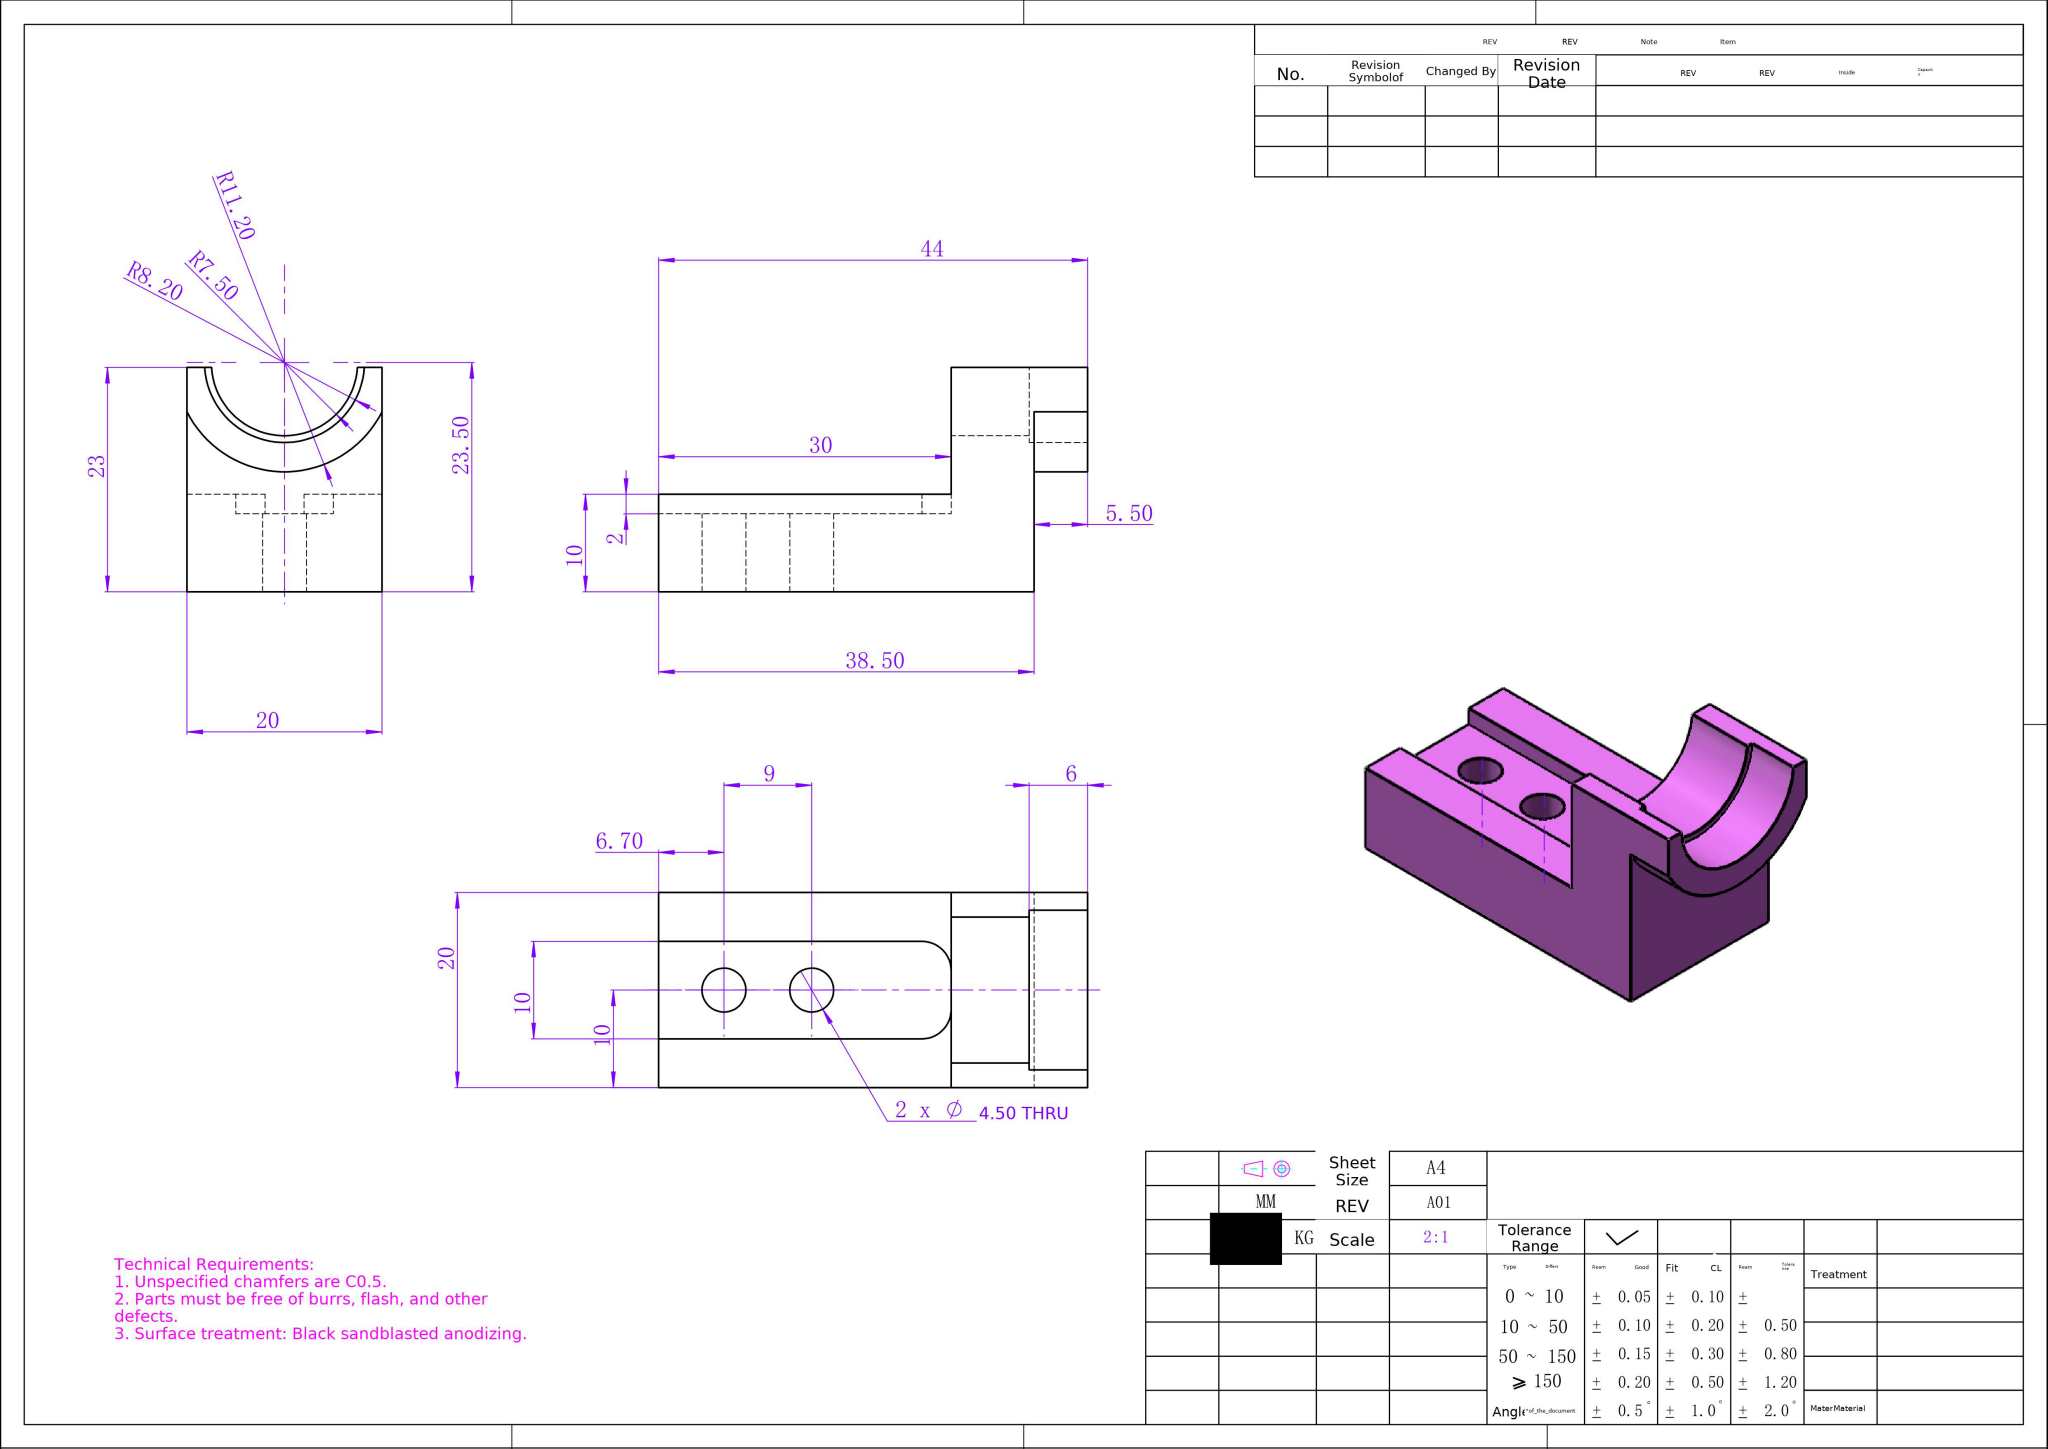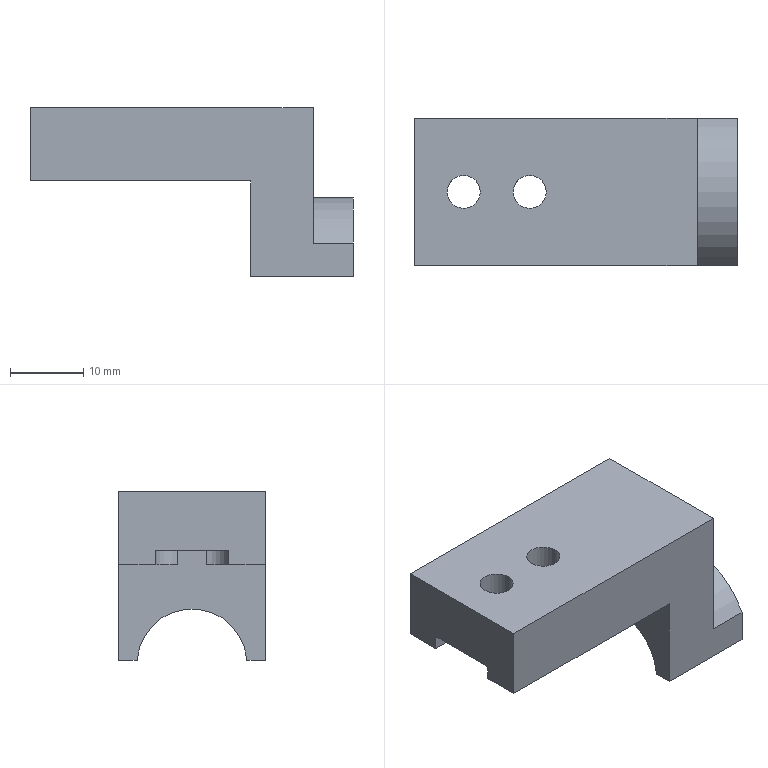Part | NX | mm | Dual-Bore Saddle Mounting Block | 1 solid | 24 faces | box 44 x 20 x 23 mm | volume 8816 mm3 | plane 15 | cylinder 9 | commonest cylinder face diameters 4.5 x4 6 x2 15 x1 16.4 x1 22.4 x1
STEP:
#1=COLOUR_RGB('',0.9529,0.498,1.);
#2=FILL_AREA_STYLE_COLOUR('',#1);
#3=FILL_AREA_STYLE('',(#2));
#4=SURFACE_STYLE_FILL_AREA(#3);
#5=SURFACE_SIDE_STYLE('',(#4));
#6=SURFACE_STYLE_USAGE(.BOTH.,#5);
#7=PRESENTATION_STYLE_ASSIGNMENT((#6));
#8=CARTESIAN_POINT('',(78.871,2.029,15.5));
#9=VERTEX_POINT('',#8);
#10=CARTESIAN_POINT('',(83.371,2.029,15.5));
#11=VERTEX_POINT('',#10);
#12=CARTESIAN_POINT('',(81.121,2.029,15.5));
#13=DIRECTION('',(0.,0.,1.));
#14=DIRECTION('',(-1.,0.,0.));
#15=AXIS2_PLACEMENT_3D('',#12,#13,#14);
#16=CIRCLE('',#15,2.25);
#17=EDGE_CURVE('',#9,#11,#16,.T.);
#18=ORIENTED_EDGE('',*,*,#17,.F.);
#19=CARTESIAN_POINT('',(78.871,2.029,23.5));
#20=VERTEX_POINT('',#19);
#21=CARTESIAN_POINT('',(78.871,2.029,23.5));
#22=DIRECTION('',(0.,0.,1.));
#23=VECTOR('',#22,1000.);
#24=LINE('',#21,#23);
#25=EDGE_CURVE('',#9,#20,#24,.T.);
#26=ORIENTED_EDGE('',*,*,#25,.T.);
#27=CARTESIAN_POINT('',(83.371,2.029,23.5));
#28=VERTEX_POINT('',#27);
#29=CARTESIAN_POINT('',(81.121,2.029,23.5));
#30=DIRECTION('',(0.,0.,1.));
#31=DIRECTION('',(1.,0.,0.));
#32=AXIS2_PLACEMENT_3D('',#29,#30,#31);
#33=CIRCLE('',#32,2.25);
#34=EDGE_CURVE('',#20,#28,#33,.T.);
#35=ORIENTED_EDGE('',*,*,#34,.T.);
#36=CARTESIAN_POINT('',(83.371,2.029,23.5));
#37=DIRECTION('',(0.,0.,1.));
#38=VECTOR('',#37,1000.);
#39=LINE('',#36,#38);
#40=EDGE_CURVE('',#11,#28,#39,.T.);
#41=ORIENTED_EDGE('',*,*,#40,.F.);
#42=EDGE_LOOP('',(#18,#26,#35,#41));
#43=FACE_OUTER_BOUND('',#42,.T.);
#44=CARTESIAN_POINT('',(81.121,2.029,23.5));
#45=DIRECTION('',(0.,0.,1.));
#46=DIRECTION('',(1.,0.,0.));
#47=AXIS2_PLACEMENT_3D('',#44,#45,#46);
#48=CYLINDRICAL_SURFACE('',#47,2.25);
#49=ADVANCED_FACE('',(#43),#48,.F.);
#50=CARTESIAN_POINT('',(87.871,2.029,15.5));
#51=VERTEX_POINT('',#50);
#52=CARTESIAN_POINT('',(92.371,2.029,15.5));
#53=VERTEX_POINT('',#52);
#54=CARTESIAN_POINT('',(90.121,2.029,15.5));
#55=DIRECTION('',(0.,0.,1.));
#56=DIRECTION('',(-1.,0.,0.));
#57=AXIS2_PLACEMENT_3D('',#54,#55,#56);
#58=CIRCLE('',#57,2.25);
#59=EDGE_CURVE('',#51,#53,#58,.T.);
#60=ORIENTED_EDGE('',*,*,#59,.F.);
#61=CARTESIAN_POINT('',(87.871,2.029,23.5));
#62=VERTEX_POINT('',#61);
#63=CARTESIAN_POINT('',(87.871,2.029,23.5));
#64=DIRECTION('',(0.,0.,1.));
#65=VECTOR('',#64,1000.);
#66=LINE('',#63,#65);
#67=EDGE_CURVE('',#51,#62,#66,.T.);
#68=ORIENTED_EDGE('',*,*,#67,.T.);
#69=CARTESIAN_POINT('',(92.371,2.029,23.5));
#70=VERTEX_POINT('',#69);
#71=CARTESIAN_POINT('',(90.121,2.029,23.5));
#72=DIRECTION('',(0.,0.,1.));
#73=DIRECTION('',(1.,0.,0.));
#74=AXIS2_PLACEMENT_3D('',#71,#72,#73);
#75=CIRCLE('',#74,2.25);
#76=EDGE_CURVE('',#62,#70,#75,.T.);
#77=ORIENTED_EDGE('',*,*,#76,.T.);
#78=CARTESIAN_POINT('',(92.371,2.029,23.5));
#79=DIRECTION('',(0.,0.,1.));
#80=VECTOR('',#79,1000.);
#81=LINE('',#78,#80);
#82=EDGE_CURVE('',#53,#70,#81,.T.);
#83=ORIENTED_EDGE('',*,*,#82,.F.);
#84=EDGE_LOOP('',(#60,#68,#77,#83));
#85=FACE_OUTER_BOUND('',#84,.T.);
#86=CARTESIAN_POINT('',(90.121,2.029,23.5));
#87=DIRECTION('',(0.,0.,1.));
#88=DIRECTION('',(1.,0.,0.));
#89=AXIS2_PLACEMENT_3D('',#86,#87,#88);
#90=CYLINDRICAL_SURFACE('',#89,2.25);
#91=ADVANCED_FACE('',(#85),#90,.F.);
#92=CARTESIAN_POINT('',(90.121,2.029,23.5));
#93=DIRECTION('',(0.,0.,1.));
#94=DIRECTION('',(1.,0.,0.));
#95=AXIS2_PLACEMENT_3D('',#92,#93,#94);
#96=CIRCLE('',#95,2.25);
#97=EDGE_CURVE('',#70,#62,#96,.T.);
#98=ORIENTED_EDGE('',*,*,#97,.F.);
#99=ORIENTED_EDGE('',*,*,#76,.F.);
#100=EDGE_LOOP('',(#98,#99));
#101=FACE_BOUND('',#100,.T.);
#102=CARTESIAN_POINT('',(81.121,2.029,23.5));
#103=DIRECTION('',(0.,0.,1.));
#104=DIRECTION('',(1.,0.,0.));
#105=AXIS2_PLACEMENT_3D('',#102,#103,#104);
#106=CIRCLE('',#105,2.25);
#107=EDGE_CURVE('',#28,#20,#106,.T.);
#108=ORIENTED_EDGE('',*,*,#107,.F.);
#109=ORIENTED_EDGE('',*,*,#34,.F.);
#110=EDGE_LOOP('',(#108,#109));
#111=FACE_BOUND('',#110,.T.);
#112=CARTESIAN_POINT('',(112.921,12.029,23.5));
#113=VERTEX_POINT('',#112);
#114=CARTESIAN_POINT('',(112.921,-7.971,23.5));
#115=VERTEX_POINT('',#114);
#116=CARTESIAN_POINT('',(112.921,12.029,23.5));
#117=DIRECTION('',(0.,-1.,0.));
#118=VECTOR('',#117,1000.);
#119=LINE('',#116,#118);
#120=EDGE_CURVE('',#113,#115,#119,.T.);
#121=ORIENTED_EDGE('',*,*,#120,.F.);
#122=CARTESIAN_POINT('',(74.421,12.029,23.5));
#123=VERTEX_POINT('',#122);
#124=CARTESIAN_POINT('',(74.421,12.029,23.5));
#125=DIRECTION('',(-1.,-0.,0.));
#126=VECTOR('',#125,1000.);
#127=LINE('',#124,#126);
#128=EDGE_CURVE('',#113,#123,#127,.T.);
#129=ORIENTED_EDGE('',*,*,#128,.T.);
#130=CARTESIAN_POINT('',(74.421,-7.971,23.5));
#131=VERTEX_POINT('',#130);
#132=CARTESIAN_POINT('',(74.421,-7.971,23.5));
#133=DIRECTION('',(0.,-1.,0.));
#134=VECTOR('',#133,1000.);
#135=LINE('',#132,#134);
#136=EDGE_CURVE('',#123,#131,#135,.T.);
#137=ORIENTED_EDGE('',*,*,#136,.T.);
#138=CARTESIAN_POINT('',(74.421,-7.971,23.5));
#139=DIRECTION('',(1.,0.,0.));
#140=VECTOR('',#139,1000.);
#141=LINE('',#138,#140);
#142=EDGE_CURVE('',#131,#115,#141,.T.);
#143=ORIENTED_EDGE('',*,*,#142,.T.);
#144=EDGE_LOOP('',(#121,#129,#137,#143));
#145=FACE_OUTER_BOUND('',#144,.T.);
#146=CARTESIAN_POINT('',(0.,0.,23.5));
#147=DIRECTION('',(0.,0.,-1.));
#148=DIRECTION('',(-1.,0.,0.));
#149=AXIS2_PLACEMENT_3D('',#146,#147,#148);
#150=PLANE('',#149);
#151=ADVANCED_FACE('',(#101,#111,#145),#150,.F.);
#152=CARTESIAN_POINT('',(104.421,-5.454,0.5));
#153=VERTEX_POINT('',#152);
#154=CARTESIAN_POINT('',(104.421,9.513,0.5));
#155=VERTEX_POINT('',#154);
#156=CARTESIAN_POINT('',(104.421,2.029,0.));
#157=DIRECTION('',(-1.,-0.,0.));
#158=DIRECTION('',(0.,-1.,0.));
#159=AXIS2_PLACEMENT_3D('',#156,#157,#158);
#160=CIRCLE('',#159,7.5);
#161=EDGE_CURVE('',#153,#155,#160,.T.);
#162=ORIENTED_EDGE('',*,*,#161,.T.);
#163=CARTESIAN_POINT('',(112.421,9.513,0.5));
#164=VERTEX_POINT('',#163);
#165=CARTESIAN_POINT('',(118.421,9.513,0.5));
#166=DIRECTION('',(1.,0.,0.));
#167=VECTOR('',#166,1000.);
#168=LINE('',#165,#167);
#169=EDGE_CURVE('',#155,#164,#168,.T.);
#170=ORIENTED_EDGE('',*,*,#169,.T.);
#171=CARTESIAN_POINT('',(112.421,-5.454,0.5));
#172=VERTEX_POINT('',#171);
#173=CARTESIAN_POINT('',(112.421,2.029,0.));
#174=DIRECTION('',(-1.,0.,0.));
#175=DIRECTION('',(0.,0.,-1.));
#176=AXIS2_PLACEMENT_3D('',#173,#174,#175);
#177=CIRCLE('',#176,7.5);
#178=EDGE_CURVE('',#172,#164,#177,.T.);
#179=ORIENTED_EDGE('',*,*,#178,.F.);
#180=CARTESIAN_POINT('',(118.421,-5.454,0.5));
#181=DIRECTION('',(-1.,-0.,0.));
#182=VECTOR('',#181,1000.);
#183=LINE('',#180,#182);
#184=EDGE_CURVE('',#172,#153,#183,.T.);
#185=ORIENTED_EDGE('',*,*,#184,.T.);
#186=EDGE_LOOP('',(#162,#170,#179,#185));
#187=FACE_OUTER_BOUND('',#186,.T.);
#188=CARTESIAN_POINT('',(118.421,2.029,0.));
#189=DIRECTION('',(-1.,-0.,0.));
#190=DIRECTION('',(0.,-1.,0.));
#191=AXIS2_PLACEMENT_3D('',#188,#189,#190);
#192=CYLINDRICAL_SURFACE('',#191,7.5);
#193=ADVANCED_FACE('',(#187),#192,.F.);
#194=CARTESIAN_POINT('',(74.421,-7.971,13.5));
#195=VERTEX_POINT('',#194);
#196=CARTESIAN_POINT('',(74.421,-2.971,13.5));
#197=VERTEX_POINT('',#196);
#198=CARTESIAN_POINT('',(74.421,-7.971,13.5));
#199=DIRECTION('',(-0.,1.,0.));
#200=VECTOR('',#199,1000.);
#201=LINE('',#198,#200);
#202=EDGE_CURVE('',#195,#197,#201,.T.);
#203=ORIENTED_EDGE('',*,*,#202,.T.);
#204=CARTESIAN_POINT('',(101.421,-2.971,13.5));
#205=VERTEX_POINT('',#204);
#206=CARTESIAN_POINT('',(74.421,-2.971,13.5));
#207=DIRECTION('',(-1.,0.,0.));
#208=VECTOR('',#207,1000.);
#209=LINE('',#206,#208);
#210=EDGE_CURVE('',#205,#197,#209,.T.);
#211=ORIENTED_EDGE('',*,*,#210,.F.);
#212=CARTESIAN_POINT('',(104.421,0.02923,13.5));
#213=VERTEX_POINT('',#212);
#214=CARTESIAN_POINT('',(101.421,0.02923,13.5));
#215=DIRECTION('',(0.,0.,-1.));
#216=DIRECTION('',(-1.,0.,0.));
#217=AXIS2_PLACEMENT_3D('',#214,#215,#216);
#218=CIRCLE('',#217,3.);
#219=EDGE_CURVE('',#213,#205,#218,.T.);
#220=ORIENTED_EDGE('',*,*,#219,.F.);
#221=CARTESIAN_POINT('',(104.421,-7.971,13.5));
#222=VERTEX_POINT('',#221);
#223=CARTESIAN_POINT('',(104.421,-7.971,13.5));
#224=DIRECTION('',(-0.,1.,0.));
#225=VECTOR('',#224,1000.);
#226=LINE('',#223,#225);
#227=EDGE_CURVE('',#222,#213,#226,.T.);
#228=ORIENTED_EDGE('',*,*,#227,.F.);
#229=CARTESIAN_POINT('',(74.421,-7.971,13.5));
#230=DIRECTION('',(1.,0.,0.));
#231=VECTOR('',#230,1000.);
#232=LINE('',#229,#231);
#233=EDGE_CURVE('',#195,#222,#232,.T.);
#234=ORIENTED_EDGE('',*,*,#233,.F.);
#235=EDGE_LOOP('',(#203,#211,#220,#228,#234));
#236=FACE_OUTER_BOUND('',#235,.T.);
#237=CARTESIAN_POINT('',(74.421,-7.971,13.5));
#238=DIRECTION('',(0.,0.,1.));
#239=DIRECTION('',(1.,0.,0.));
#240=AXIS2_PLACEMENT_3D('',#237,#238,#239);
#241=PLANE('',#240);
#242=ADVANCED_FACE('',(#236),#241,.F.);
#243=ORIENTED_EDGE('',*,*,#67,.F.);
#244=CARTESIAN_POINT('',(90.121,2.029,15.5));
#245=DIRECTION('',(0.,0.,1.));
#246=DIRECTION('',(-1.,0.,0.));
#247=AXIS2_PLACEMENT_3D('',#244,#245,#246);
#248=CIRCLE('',#247,2.25);
#249=EDGE_CURVE('',#53,#51,#248,.T.);
#250=ORIENTED_EDGE('',*,*,#249,.F.);
#251=ORIENTED_EDGE('',*,*,#82,.T.);
#252=ORIENTED_EDGE('',*,*,#97,.T.);
#253=EDGE_LOOP('',(#243,#250,#251,#252));
#254=FACE_OUTER_BOUND('',#253,.T.);
#255=CARTESIAN_POINT('',(90.121,2.029,23.5));
#256=DIRECTION('',(0.,0.,1.));
#257=DIRECTION('',(1.,0.,0.));
#258=AXIS2_PLACEMENT_3D('',#255,#256,#257);
#259=CYLINDRICAL_SURFACE('',#258,2.25);
#260=ADVANCED_FACE('',(#254),#259,.F.);
#261=ORIENTED_EDGE('',*,*,#25,.F.);
#262=CARTESIAN_POINT('',(81.121,2.029,15.5));
#263=DIRECTION('',(0.,0.,1.));
#264=DIRECTION('',(-1.,0.,0.));
#265=AXIS2_PLACEMENT_3D('',#262,#263,#264);
#266=CIRCLE('',#265,2.25);
#267=EDGE_CURVE('',#11,#9,#266,.T.);
#268=ORIENTED_EDGE('',*,*,#267,.F.);
#269=ORIENTED_EDGE('',*,*,#40,.T.);
#270=ORIENTED_EDGE('',*,*,#107,.T.);
#271=EDGE_LOOP('',(#261,#268,#269,#270));
#272=FACE_OUTER_BOUND('',#271,.T.);
#273=CARTESIAN_POINT('',(81.121,2.029,23.5));
#274=DIRECTION('',(0.,0.,1.));
#275=DIRECTION('',(1.,0.,0.));
#276=AXIS2_PLACEMENT_3D('',#273,#274,#275);
#277=CYLINDRICAL_SURFACE('',#276,2.25);
#278=ADVANCED_FACE('',(#272),#277,.F.);
#279=CARTESIAN_POINT('',(118.421,-7.971,5.044));
#280=VERTEX_POINT('',#279);
#281=CARTESIAN_POINT('',(118.421,-7.971,0.5));
#282=VERTEX_POINT('',#281);
#283=CARTESIAN_POINT('',(118.421,-7.971,23.5));
#284=DIRECTION('',(0.,0.,-1.));
#285=VECTOR('',#284,1000.);
#286=LINE('',#283,#285);
#287=EDGE_CURVE('',#280,#282,#286,.T.);
#288=ORIENTED_EDGE('',*,*,#287,.T.);
#289=CARTESIAN_POINT('',(118.421,-6.156,0.5));
#290=VERTEX_POINT('',#289);
#291=CARTESIAN_POINT('',(118.421,-7.971,0.5));
#292=DIRECTION('',(0.,1.,0.));
#293=VECTOR('',#292,1000.);
#294=LINE('',#291,#293);
#295=EDGE_CURVE('',#282,#290,#294,.T.);
#296=ORIENTED_EDGE('',*,*,#295,.T.);
#297=CARTESIAN_POINT('',(118.421,10.214,0.5));
#298=VERTEX_POINT('',#297);
#299=CARTESIAN_POINT('',(118.421,2.029,0.));
#300=DIRECTION('',(1.,0.,0.));
#301=DIRECTION('',(0.,0.,-1.));
#302=AXIS2_PLACEMENT_3D('',#299,#300,#301);
#303=CIRCLE('',#302,8.2);
#304=EDGE_CURVE('',#298,#290,#303,.T.);
#305=ORIENTED_EDGE('',*,*,#304,.F.);
#306=CARTESIAN_POINT('',(118.421,12.029,0.5));
#307=VERTEX_POINT('',#306);
#308=CARTESIAN_POINT('',(118.421,-7.971,0.5));
#309=DIRECTION('',(0.,1.,0.));
#310=VECTOR('',#309,1000.);
#311=LINE('',#308,#310);
#312=EDGE_CURVE('',#298,#307,#311,.T.);
#313=ORIENTED_EDGE('',*,*,#312,.T.);
#314=CARTESIAN_POINT('',(118.421,12.029,5.044));
#315=VERTEX_POINT('',#314);
#316=CARTESIAN_POINT('',(118.421,12.029,23.5));
#317=DIRECTION('',(0.,0.,-1.));
#318=VECTOR('',#317,1000.);
#319=LINE('',#316,#318);
#320=EDGE_CURVE('',#315,#307,#319,.T.);
#321=ORIENTED_EDGE('',*,*,#320,.F.);
#322=CARTESIAN_POINT('',(118.421,2.029,0.));
#323=DIRECTION('',(-1.,0.,0.));
#324=DIRECTION('',(0.,0.,-1.));
#325=AXIS2_PLACEMENT_3D('',#322,#323,#324);
#326=CIRCLE('',#325,11.2);
#327=EDGE_CURVE('',#280,#315,#326,.T.);
#328=ORIENTED_EDGE('',*,*,#327,.F.);
#329=EDGE_LOOP('',(#288,#296,#305,#313,#321,#328));
#330=FACE_OUTER_BOUND('',#329,.T.);
#331=CARTESIAN_POINT('',(118.421,-7.971,23.5));
#332=DIRECTION('',(-1.,0.,0.));
#333=DIRECTION('',(0.,0.,1.));
#334=AXIS2_PLACEMENT_3D('',#331,#332,#333);
#335=PLANE('',#334);
#336=ADVANCED_FACE('',(#330),#335,.F.);
#337=ORIENTED_EDGE('',*,*,#320,.T.);
#338=CARTESIAN_POINT('',(104.421,12.029,0.5));
#339=VERTEX_POINT('',#338);
#340=CARTESIAN_POINT('',(118.421,12.029,0.5));
#341=DIRECTION('',(-1.,-0.,0.));
#342=VECTOR('',#341,1000.);
#343=LINE('',#340,#342);
#344=EDGE_CURVE('',#307,#339,#343,.T.);
#345=ORIENTED_EDGE('',*,*,#344,.T.);
#346=CARTESIAN_POINT('',(104.421,12.029,13.5));
#347=VERTEX_POINT('',#346);
#348=CARTESIAN_POINT('',(104.421,12.029,0.));
#349=DIRECTION('',(0.,0.,-1.));
#350=VECTOR('',#349,1000.);
#351=LINE('',#348,#350);
#352=EDGE_CURVE('',#347,#339,#351,.T.);
#353=ORIENTED_EDGE('',*,*,#352,.F.);
#354=CARTESIAN_POINT('',(74.421,12.029,13.5));
#355=VERTEX_POINT('',#354);
#356=CARTESIAN_POINT('',(74.421,12.029,13.5));
#357=DIRECTION('',(1.,0.,0.));
#358=VECTOR('',#357,1000.);
#359=LINE('',#356,#358);
#360=EDGE_CURVE('',#355,#347,#359,.T.);
#361=ORIENTED_EDGE('',*,*,#360,.F.);
#362=CARTESIAN_POINT('',(74.421,12.029,23.5));
#363=DIRECTION('',(0.,0.,-1.));
#364=VECTOR('',#363,1000.);
#365=LINE('',#362,#364);
#366=EDGE_CURVE('',#123,#355,#365,.T.);
#367=ORIENTED_EDGE('',*,*,#366,.F.);
#368=ORIENTED_EDGE('',*,*,#128,.F.);
#369=CARTESIAN_POINT('',(112.921,12.029,5.044));
#370=VERTEX_POINT('',#369);
#371=CARTESIAN_POINT('',(112.921,12.029,23.5));
#372=DIRECTION('',(0.,0.,1.));
#373=VECTOR('',#372,1000.);
#374=LINE('',#371,#373);
#375=EDGE_CURVE('',#370,#113,#374,.T.);
#376=ORIENTED_EDGE('',*,*,#375,.F.);
#377=CARTESIAN_POINT('',(112.921,12.029,5.044));
#378=DIRECTION('',(1.,0.,0.));
#379=VECTOR('',#378,1000.);
#380=LINE('',#377,#379);
#381=EDGE_CURVE('',#370,#315,#380,.T.);
#382=ORIENTED_EDGE('',*,*,#381,.T.);
#383=EDGE_LOOP('',(#337,#345,#353,#361,#367,#368,#376,#382));
#384=FACE_OUTER_BOUND('',#383,.T.);
#385=CARTESIAN_POINT('',(74.421,12.029,23.5));
#386=DIRECTION('',(0.,-1.,0.));
#387=DIRECTION('',(1.,0.,0.));
#388=AXIS2_PLACEMENT_3D('',#385,#386,#387);
#389=PLANE('',#388);
#390=ADVANCED_FACE('',(#384),#389,.F.);
#391=CARTESIAN_POINT('',(74.421,-2.971,15.5));
#392=VERTEX_POINT('',#391);
#393=CARTESIAN_POINT('',(74.421,7.029,15.5));
#394=VERTEX_POINT('',#393);
#395=CARTESIAN_POINT('',(74.421,7.029,15.5));
#396=DIRECTION('',(0.,1.,0.));
#397=VECTOR('',#396,1000.);
#398=LINE('',#395,#397);
#399=EDGE_CURVE('',#392,#394,#398,.T.);
#400=ORIENTED_EDGE('',*,*,#399,.F.);
#401=CARTESIAN_POINT('',(74.421,-2.971,15.5));
#402=DIRECTION('',(0.,0.,-1.));
#403=VECTOR('',#402,1000.);
#404=LINE('',#401,#403);
#405=EDGE_CURVE('',#392,#197,#404,.T.);
#406=ORIENTED_EDGE('',*,*,#405,.T.);
#407=ORIENTED_EDGE('',*,*,#202,.F.);
#408=CARTESIAN_POINT('',(74.421,-7.971,23.5));
#409=DIRECTION('',(0.,0.,-1.));
#410=VECTOR('',#409,1000.);
#411=LINE('',#408,#410);
#412=EDGE_CURVE('',#131,#195,#411,.T.);
#413=ORIENTED_EDGE('',*,*,#412,.F.);
#414=ORIENTED_EDGE('',*,*,#136,.F.);
#415=ORIENTED_EDGE('',*,*,#366,.T.);
#416=CARTESIAN_POINT('',(74.421,7.029,13.5));
#417=VERTEX_POINT('',#416);
#418=CARTESIAN_POINT('',(74.421,-7.971,13.5));
#419=DIRECTION('',(-0.,1.,0.));
#420=VECTOR('',#419,1000.);
#421=LINE('',#418,#420);
#422=EDGE_CURVE('',#417,#355,#421,.T.);
#423=ORIENTED_EDGE('',*,*,#422,.F.);
#424=CARTESIAN_POINT('',(74.421,7.029,15.5));
#425=DIRECTION('',(0.,0.,-1.));
#426=VECTOR('',#425,1000.);
#427=LINE('',#424,#426);
#428=EDGE_CURVE('',#394,#417,#427,.T.);
#429=ORIENTED_EDGE('',*,*,#428,.F.);
#430=EDGE_LOOP('',(#400,#406,#407,#413,#414,#415,#423,#429));
#431=FACE_OUTER_BOUND('',#430,.T.);
#432=CARTESIAN_POINT('',(74.421,-7.971,23.5));
#433=DIRECTION('',(1.,0.,0.));
#434=DIRECTION('',(0.,0.,-1.));
#435=AXIS2_PLACEMENT_3D('',#432,#433,#434);
#436=PLANE('',#435);
#437=ADVANCED_FACE('',(#431),#436,.F.);
#438=CARTESIAN_POINT('',(104.421,-7.971,0.5));
#439=VERTEX_POINT('',#438);
#440=CARTESIAN_POINT('',(104.421,-7.971,0.));
#441=DIRECTION('',(0.,0.,-1.));
#442=VECTOR('',#441,1000.);
#443=LINE('',#440,#442);
#444=EDGE_CURVE('',#222,#439,#443,.T.);
#445=ORIENTED_EDGE('',*,*,#444,.T.);
#446=CARTESIAN_POINT('',(118.421,-7.971,0.5));
#447=DIRECTION('',(-1.,-0.,0.));
#448=VECTOR('',#447,1000.);
#449=LINE('',#446,#448);
#450=EDGE_CURVE('',#282,#439,#449,.T.);
#451=ORIENTED_EDGE('',*,*,#450,.F.);
#452=ORIENTED_EDGE('',*,*,#287,.F.);
#453=CARTESIAN_POINT('',(112.921,-7.971,5.044));
#454=VERTEX_POINT('',#453);
#455=CARTESIAN_POINT('',(112.921,-7.971,5.044));
#456=DIRECTION('',(1.,0.,0.));
#457=VECTOR('',#456,1000.);
#458=LINE('',#455,#457);
#459=EDGE_CURVE('',#454,#280,#458,.T.);
#460=ORIENTED_EDGE('',*,*,#459,.F.);
#461=CARTESIAN_POINT('',(112.921,-7.971,23.5));
#462=DIRECTION('',(0.,0.,-1.));
#463=VECTOR('',#462,1000.);
#464=LINE('',#461,#463);
#465=EDGE_CURVE('',#115,#454,#464,.T.);
#466=ORIENTED_EDGE('',*,*,#465,.F.);
#467=ORIENTED_EDGE('',*,*,#142,.F.);
#468=ORIENTED_EDGE('',*,*,#412,.T.);
#469=ORIENTED_EDGE('',*,*,#233,.T.);
#470=EDGE_LOOP('',(#445,#451,#452,#460,#466,#467,#468,#469));
#471=FACE_OUTER_BOUND('',#470,.T.);
#472=CARTESIAN_POINT('',(74.421,-7.971,23.5));
#473=DIRECTION('',(0.,1.,0.));
#474=DIRECTION('',(0.,0.,1.));
#475=AXIS2_PLACEMENT_3D('',#472,#473,#474);
#476=PLANE('',#475);
#477=ADVANCED_FACE('',(#471),#476,.F.);
#478=ORIENTED_EDGE('',*,*,#352,.T.);
#479=CARTESIAN_POINT('',(104.421,-7.971,0.5));
#480=DIRECTION('',(0.,1.,0.));
#481=VECTOR('',#480,1000.);
#482=LINE('',#479,#481);
#483=EDGE_CURVE('',#155,#339,#482,.T.);
#484=ORIENTED_EDGE('',*,*,#483,.F.);
#485=ORIENTED_EDGE('',*,*,#161,.F.);
#486=CARTESIAN_POINT('',(104.421,-7.971,0.5));
#487=DIRECTION('',(0.,1.,0.));
#488=VECTOR('',#487,1000.);
#489=LINE('',#486,#488);
#490=EDGE_CURVE('',#439,#153,#489,.T.);
#491=ORIENTED_EDGE('',*,*,#490,.F.);
#492=ORIENTED_EDGE('',*,*,#444,.F.);
#493=ORIENTED_EDGE('',*,*,#227,.T.);
#494=CARTESIAN_POINT('',(104.421,0.02923,15.5));
#495=VERTEX_POINT('',#494);
#496=CARTESIAN_POINT('',(104.421,0.02923,15.5));
#497=DIRECTION('',(0.,0.,-1.));
#498=VECTOR('',#497,1000.);
#499=LINE('',#496,#498);
#500=EDGE_CURVE('',#495,#213,#499,.T.);
#501=ORIENTED_EDGE('',*,*,#500,.F.);
#502=CARTESIAN_POINT('',(104.421,4.029,15.5));
#503=VERTEX_POINT('',#502);
#504=CARTESIAN_POINT('',(104.421,4.029,15.5));
#505=DIRECTION('',(0.,-1.,0.));
#506=VECTOR('',#505,1000.);
#507=LINE('',#504,#506);
#508=EDGE_CURVE('',#503,#495,#507,.T.);
#509=ORIENTED_EDGE('',*,*,#508,.F.);
#510=CARTESIAN_POINT('',(104.421,4.029,13.5));
#511=VERTEX_POINT('',#510);
#512=CARTESIAN_POINT('',(104.421,4.029,15.5));
#513=DIRECTION('',(0.,0.,-1.));
#514=VECTOR('',#513,1000.);
#515=LINE('',#512,#514);
#516=EDGE_CURVE('',#503,#511,#515,.T.);
#517=ORIENTED_EDGE('',*,*,#516,.T.);
#518=CARTESIAN_POINT('',(104.421,-7.971,13.5));
#519=DIRECTION('',(-0.,1.,0.));
#520=VECTOR('',#519,1000.);
#521=LINE('',#518,#520);
#522=EDGE_CURVE('',#511,#347,#521,.T.);
#523=ORIENTED_EDGE('',*,*,#522,.T.);
#524=EDGE_LOOP('',(#478,#484,#485,#491,#492,#493,#501,#509,#517,#523));
#525=FACE_OUTER_BOUND('',#524,.T.);
#526=CARTESIAN_POINT('',(104.421,-7.971,0.));
#527=DIRECTION('',(1.,0.,0.));
#528=DIRECTION('',(-0.,1.,0.));
#529=AXIS2_PLACEMENT_3D('',#526,#527,#528);
#530=PLANE('',#529);
#531=ADVANCED_FACE('',(#525),#530,.F.);
#532=ORIENTED_EDGE('',*,*,#522,.F.);
#533=CARTESIAN_POINT('',(101.421,7.029,13.5));
#534=VERTEX_POINT('',#533);
#535=CARTESIAN_POINT('',(101.421,4.029,13.5));
#536=DIRECTION('',(0.,0.,-1.));
#537=DIRECTION('',(-1.,0.,0.));
#538=AXIS2_PLACEMENT_3D('',#535,#536,#537);
#539=CIRCLE('',#538,3.);
#540=EDGE_CURVE('',#534,#511,#539,.T.);
#541=ORIENTED_EDGE('',*,*,#540,.F.);
#542=CARTESIAN_POINT('',(74.421,7.029,13.5));
#543=DIRECTION('',(1.,-0.,0.));
#544=VECTOR('',#543,1000.);
#545=LINE('',#542,#544);
#546=EDGE_CURVE('',#417,#534,#545,.T.);
#547=ORIENTED_EDGE('',*,*,#546,.F.);
#548=ORIENTED_EDGE('',*,*,#422,.T.);
#549=ORIENTED_EDGE('',*,*,#360,.T.);
#550=EDGE_LOOP('',(#532,#541,#547,#548,#549));
#551=FACE_OUTER_BOUND('',#550,.T.);
#552=CARTESIAN_POINT('',(74.421,-7.971,13.5));
#553=DIRECTION('',(0.,0.,1.));
#554=DIRECTION('',(1.,0.,0.));
#555=AXIS2_PLACEMENT_3D('',#552,#553,#554);
#556=PLANE('',#555);
#557=ADVANCED_FACE('',(#551),#556,.F.);
#558=ORIENTED_EDGE('',*,*,#399,.T.);
#559=CARTESIAN_POINT('',(101.421,7.029,15.5));
#560=VERTEX_POINT('',#559);
#561=CARTESIAN_POINT('',(74.421,7.029,15.5));
#562=DIRECTION('',(1.,-0.,0.));
#563=VECTOR('',#562,1000.);
#564=LINE('',#561,#563);
#565=EDGE_CURVE('',#394,#560,#564,.T.);
#566=ORIENTED_EDGE('',*,*,#565,.T.);
#567=CARTESIAN_POINT('',(101.421,4.029,15.5));
#568=DIRECTION('',(0.,0.,-1.));
#569=DIRECTION('',(-1.,0.,0.));
#570=AXIS2_PLACEMENT_3D('',#567,#568,#569);
#571=CIRCLE('',#570,3.);
#572=EDGE_CURVE('',#560,#503,#571,.T.);
#573=ORIENTED_EDGE('',*,*,#572,.T.);
#574=ORIENTED_EDGE('',*,*,#508,.T.);
#575=CARTESIAN_POINT('',(101.421,-2.971,15.5));
#576=VERTEX_POINT('',#575);
#577=CARTESIAN_POINT('',(101.421,0.02923,15.5));
#578=DIRECTION('',(0.,0.,-1.));
#579=DIRECTION('',(-1.,0.,0.));
#580=AXIS2_PLACEMENT_3D('',#577,#578,#579);
#581=CIRCLE('',#580,3.);
#582=EDGE_CURVE('',#495,#576,#581,.T.);
#583=ORIENTED_EDGE('',*,*,#582,.T.);
#584=CARTESIAN_POINT('',(74.421,-2.971,15.5));
#585=DIRECTION('',(-1.,0.,0.));
#586=VECTOR('',#585,1000.);
#587=LINE('',#584,#586);
#588=EDGE_CURVE('',#576,#392,#587,.T.);
#589=ORIENTED_EDGE('',*,*,#588,.T.);
#590=EDGE_LOOP('',(#558,#566,#573,#574,#583,#589));
#591=FACE_OUTER_BOUND('',#590,.T.);
#592=ORIENTED_EDGE('',*,*,#267,.T.);
#593=ORIENTED_EDGE('',*,*,#17,.T.);
#594=EDGE_LOOP('',(#592,#593));
#595=FACE_BOUND('',#594,.T.);
#596=ORIENTED_EDGE('',*,*,#249,.T.);
#597=ORIENTED_EDGE('',*,*,#59,.T.);
#598=EDGE_LOOP('',(#596,#597));
#599=FACE_BOUND('',#598,.T.);
#600=CARTESIAN_POINT('',(101.421,0.02923,15.5));
#601=DIRECTION('',(0.,0.,-1.));
#602=DIRECTION('',(-1.,0.,0.));
#603=AXIS2_PLACEMENT_3D('',#600,#601,#602);
#604=PLANE('',#603);
#605=ADVANCED_FACE('',(#591,#595,#599),#604,.T.);
#606=ORIENTED_EDGE('',*,*,#210,.T.);
#607=ORIENTED_EDGE('',*,*,#405,.F.);
#608=ORIENTED_EDGE('',*,*,#588,.F.);
#609=CARTESIAN_POINT('',(101.421,-2.971,15.5));
#610=DIRECTION('',(0.,0.,-1.));
#611=VECTOR('',#610,1000.);
#612=LINE('',#609,#611);
#613=EDGE_CURVE('',#576,#205,#612,.T.);
#614=ORIENTED_EDGE('',*,*,#613,.T.);
#615=EDGE_LOOP('',(#606,#607,#608,#614));
#616=FACE_OUTER_BOUND('',#615,.T.);
#617=CARTESIAN_POINT('',(74.421,-2.971,15.5));
#618=DIRECTION('',(-0.,-1.,0.));
#619=DIRECTION('',(1.,-0.,0.));
#620=AXIS2_PLACEMENT_3D('',#617,#618,#619);
#621=PLANE('',#620);
#622=ADVANCED_FACE('',(#616),#621,.F.);
#623=ORIENTED_EDGE('',*,*,#219,.T.);
#624=ORIENTED_EDGE('',*,*,#613,.F.);
#625=ORIENTED_EDGE('',*,*,#582,.F.);
#626=ORIENTED_EDGE('',*,*,#500,.T.);
#627=EDGE_LOOP('',(#623,#624,#625,#626));
#628=FACE_OUTER_BOUND('',#627,.T.);
#629=CARTESIAN_POINT('',(101.421,0.02923,15.5));
#630=DIRECTION('',(0.,0.,-1.));
#631=DIRECTION('',(-1.,0.,0.));
#632=AXIS2_PLACEMENT_3D('',#629,#630,#631);
#633=CYLINDRICAL_SURFACE('',#632,3.);
#634=ADVANCED_FACE('',(#628),#633,.F.);
#635=ORIENTED_EDGE('',*,*,#540,.T.);
#636=ORIENTED_EDGE('',*,*,#516,.F.);
#637=ORIENTED_EDGE('',*,*,#572,.F.);
#638=CARTESIAN_POINT('',(101.421,7.029,15.5));
#639=DIRECTION('',(0.,0.,-1.));
#640=VECTOR('',#639,1000.);
#641=LINE('',#638,#640);
#642=EDGE_CURVE('',#560,#534,#641,.T.);
#643=ORIENTED_EDGE('',*,*,#642,.T.);
#644=EDGE_LOOP('',(#635,#636,#637,#643));
#645=FACE_OUTER_BOUND('',#644,.T.);
#646=CARTESIAN_POINT('',(101.421,4.029,15.5));
#647=DIRECTION('',(0.,0.,-1.));
#648=DIRECTION('',(-1.,0.,0.));
#649=AXIS2_PLACEMENT_3D('',#646,#647,#648);
#650=CYLINDRICAL_SURFACE('',#649,3.);
#651=ADVANCED_FACE('',(#645),#650,.F.);
#652=ORIENTED_EDGE('',*,*,#546,.T.);
#653=ORIENTED_EDGE('',*,*,#642,.F.);
#654=ORIENTED_EDGE('',*,*,#565,.F.);
#655=ORIENTED_EDGE('',*,*,#428,.T.);
#656=EDGE_LOOP('',(#652,#653,#654,#655));
#657=FACE_OUTER_BOUND('',#656,.T.);
#658=CARTESIAN_POINT('',(74.421,7.029,15.5));
#659=DIRECTION('',(0.,1.,0.));
#660=DIRECTION('',(-1.,0.,0.));
#661=AXIS2_PLACEMENT_3D('',#658,#659,#660);
#662=PLANE('',#661);
#663=ADVANCED_FACE('',(#657),#662,.F.);
#664=ORIENTED_EDGE('',*,*,#304,.T.);
#665=CARTESIAN_POINT('',(112.421,-6.156,0.5));
#666=VERTEX_POINT('',#665);
#667=CARTESIAN_POINT('',(112.421,-6.156,0.5));
#668=DIRECTION('',(-1.,0.,0.));
#669=VECTOR('',#668,1000.);
#670=LINE('',#667,#669);
#671=EDGE_CURVE('',#290,#666,#670,.T.);
#672=ORIENTED_EDGE('',*,*,#671,.T.);
#673=CARTESIAN_POINT('',(112.421,10.214,0.5));
#674=VERTEX_POINT('',#673);
#675=CARTESIAN_POINT('',(112.421,2.029,0.));
#676=DIRECTION('',(1.,0.,0.));
#677=DIRECTION('',(0.,0.,-1.));
#678=AXIS2_PLACEMENT_3D('',#675,#676,#677);
#679=CIRCLE('',#678,8.2);
#680=EDGE_CURVE('',#674,#666,#679,.T.);
#681=ORIENTED_EDGE('',*,*,#680,.F.);
#682=CARTESIAN_POINT('',(112.421,10.214,0.5));
#683=DIRECTION('',(1.,0.,0.));
#684=VECTOR('',#683,1000.);
#685=LINE('',#682,#684);
#686=EDGE_CURVE('',#674,#298,#685,.T.);
#687=ORIENTED_EDGE('',*,*,#686,.T.);
#688=EDGE_LOOP('',(#664,#672,#681,#687));
#689=FACE_OUTER_BOUND('',#688,.T.);
#690=CARTESIAN_POINT('',(112.421,2.029,0.));
#691=DIRECTION('',(1.,0.,0.));
#692=DIRECTION('',(0.,0.,-1.));
#693=AXIS2_PLACEMENT_3D('',#690,#691,#692);
#694=CYLINDRICAL_SURFACE('',#693,8.2);
#695=ADVANCED_FACE('',(#689),#694,.F.);
#696=CARTESIAN_POINT('',(112.421,2.029,0.5));
#697=DIRECTION('',(0.,-1.,-0.));
#698=VECTOR('',#697,1000.);
#699=LINE('',#696,#698);
#700=EDGE_CURVE('',#674,#164,#699,.T.);
#701=ORIENTED_EDGE('',*,*,#700,.F.);
#702=ORIENTED_EDGE('',*,*,#680,.T.);
#703=CARTESIAN_POINT('',(112.421,2.029,0.5));
#704=DIRECTION('',(0.,-1.,-0.));
#705=VECTOR('',#704,1000.);
#706=LINE('',#703,#705);
#707=EDGE_CURVE('',#172,#666,#706,.T.);
#708=ORIENTED_EDGE('',*,*,#707,.F.);
#709=ORIENTED_EDGE('',*,*,#178,.T.);
#710=EDGE_LOOP('',(#701,#702,#708,#709));
#711=FACE_OUTER_BOUND('',#710,.T.);
#712=CARTESIAN_POINT('',(112.421,2.029,0.));
#713=DIRECTION('',(1.,0.,0.));
#714=DIRECTION('',(0.,0.,-1.));
#715=AXIS2_PLACEMENT_3D('',#712,#713,#714);
#716=PLANE('',#715);
#717=ADVANCED_FACE('',(#711),#716,.T.);
#718=ORIENTED_EDGE('',*,*,#327,.T.);
#719=ORIENTED_EDGE('',*,*,#381,.F.);
#720=CARTESIAN_POINT('',(112.921,2.029,0.));
#721=DIRECTION('',(-1.,0.,0.));
#722=DIRECTION('',(0.,0.,-1.));
#723=AXIS2_PLACEMENT_3D('',#720,#721,#722);
#724=CIRCLE('',#723,11.2);
#725=EDGE_CURVE('',#454,#370,#724,.T.);
#726=ORIENTED_EDGE('',*,*,#725,.F.);
#727=ORIENTED_EDGE('',*,*,#459,.T.);
#728=EDGE_LOOP('',(#718,#719,#726,#727));
#729=FACE_OUTER_BOUND('',#728,.T.);
#730=CARTESIAN_POINT('',(112.921,2.029,0.));
#731=DIRECTION('',(1.,0.,0.));
#732=DIRECTION('',(0.,0.,-1.));
#733=AXIS2_PLACEMENT_3D('',#730,#731,#732);
#734=CYLINDRICAL_SURFACE('',#733,11.2);
#735=ADVANCED_FACE('',(#729),#734,.T.);
#736=ORIENTED_EDGE('',*,*,#120,.T.);
#737=ORIENTED_EDGE('',*,*,#465,.T.);
#738=ORIENTED_EDGE('',*,*,#725,.T.);
#739=ORIENTED_EDGE('',*,*,#375,.T.);
#740=EDGE_LOOP('',(#736,#737,#738,#739));
#741=FACE_OUTER_BOUND('',#740,.T.);
#742=CARTESIAN_POINT('',(112.921,2.029,0.));
#743=DIRECTION('',(1.,0.,0.));
#744=DIRECTION('',(0.,0.,-1.));
#745=AXIS2_PLACEMENT_3D('',#742,#743,#744);
#746=PLANE('',#745);
#747=ADVANCED_FACE('',(#741),#746,.T.);
#748=ORIENTED_EDGE('',*,*,#707,.T.);
#749=ORIENTED_EDGE('',*,*,#671,.F.);
#750=ORIENTED_EDGE('',*,*,#295,.F.);
#751=ORIENTED_EDGE('',*,*,#450,.T.);
#752=ORIENTED_EDGE('',*,*,#490,.T.);
#753=ORIENTED_EDGE('',*,*,#184,.F.);
#754=EDGE_LOOP('',(#748,#749,#750,#751,#752,#753));
#755=FACE_OUTER_BOUND('',#754,.T.);
#756=CARTESIAN_POINT('',(118.421,-7.971,0.5));
#757=DIRECTION('',(0.,-0.,1.));
#758=DIRECTION('',(0.,-1.,-0.));
#759=AXIS2_PLACEMENT_3D('',#756,#757,#758);
#760=PLANE('',#759);
#761=ADVANCED_FACE('',(#755),#760,.F.);
#762=ORIENTED_EDGE('',*,*,#483,.T.);
#763=ORIENTED_EDGE('',*,*,#344,.F.);
#764=ORIENTED_EDGE('',*,*,#312,.F.);
#765=ORIENTED_EDGE('',*,*,#686,.F.);
#766=ORIENTED_EDGE('',*,*,#700,.T.);
#767=ORIENTED_EDGE('',*,*,#169,.F.);
#768=EDGE_LOOP('',(#762,#763,#764,#765,#766,#767));
#769=FACE_OUTER_BOUND('',#768,.T.);
#770=CARTESIAN_POINT('',(118.421,-7.971,0.5));
#771=DIRECTION('',(0.,-0.,1.));
#772=DIRECTION('',(0.,-1.,-0.));
#773=AXIS2_PLACEMENT_3D('',#770,#771,#772);
#774=PLANE('',#773);
#775=ADVANCED_FACE('',(#769),#774,.F.);
#776=CLOSED_SHELL('',(#49,#91,#151,#193,#242,#260,#278,#336,#390,#437,#477,#531,#557,#605,#622,#634,#651,#663,#695,#717,#735,#747,#761,#775));
#777=MANIFOLD_SOLID_BREP('',#776);
#778=STYLED_ITEM('',(#7),#777);
#779=PRESENTATION_LAYER_ASSIGNMENT('','',(#778));
#780=COLOUR_RGB('',0.9529,0.498,1.);
#781=FILL_AREA_STYLE_COLOUR('',#780);
#782=FILL_AREA_STYLE('',(#781));
#783=SURFACE_STYLE_FILL_AREA(#782);
#784=SURFACE_SIDE_STYLE('',(#783));
#785=SURFACE_STYLE_USAGE(.BOTH.,#784);
#786=PRESENTATION_STYLE_ASSIGNMENT((#785));
#787=CARTESIAN_POINT('',(0.,0.,0.));
#788=DIRECTION('',(0.,0.,1.));
#789=DIRECTION('',(1.,0.,0.));
#790=AXIS2_PLACEMENT_3D('',#787,#788,#789);
#791=(LENGTH_UNIT()NAMED_UNIT(*)SI_UNIT(.MILLI.,.METRE.));
#792=UNCERTAINTY_MEASURE_WITH_UNIT(LENGTH_MEASURE(0.00001),#791,'','');
#793=(NAMED_UNIT(*)PLANE_ANGLE_UNIT()SI_UNIT($,.RADIAN.));
#794=(NAMED_UNIT(*)SI_UNIT($,.STERADIAN.)SOLID_ANGLE_UNIT());
#795=(GEOMETRIC_REPRESENTATION_CONTEXT(3)GLOBAL_UNCERTAINTY_ASSIGNED_CONTEXT((#792))GLOBAL_UNIT_ASSIGNED_CONTEXT((#791,#793,#794))REPRESENTATION_CONTEXT('',''));
#796=ADVANCED_BREP_SHAPE_REPRESENTATION('',(#777,#790),#795);
#797=STYLED_ITEM('',(#786),#796);
#798=PRESENTATION_LAYER_ASSIGNMENT('','',(#797));
#799=(LENGTH_UNIT()NAMED_UNIT(*)SI_UNIT(.MILLI.,.METRE.));
#800=UNCERTAINTY_MEASURE_WITH_UNIT(LENGTH_MEASURE(0.00001),#799,'','');
#801=(NAMED_UNIT(*)PLANE_ANGLE_UNIT()SI_UNIT($,.RADIAN.));
#802=(NAMED_UNIT(*)SI_UNIT($,.STERADIAN.)SOLID_ANGLE_UNIT());
#803=(GEOMETRIC_REPRESENTATION_CONTEXT(3)GLOBAL_UNCERTAINTY_ASSIGNED_CONTEXT((#800))GLOBAL_UNIT_ASSIGNED_CONTEXT((#799,#801,#802))REPRESENTATION_CONTEXT('',''));
#804=MECHANICAL_DESIGN_GEOMETRIC_PRESENTATION_REPRESENTATION('',(#797),#803);
#805=(LENGTH_UNIT()NAMED_UNIT(*)SI_UNIT(.MILLI.,.METRE.));
#806=UNCERTAINTY_MEASURE_WITH_UNIT(LENGTH_MEASURE(0.00001),#805,'','');
#807=(NAMED_UNIT(*)PLANE_ANGLE_UNIT()SI_UNIT($,.RADIAN.));
#808=(NAMED_UNIT(*)SI_UNIT($,.STERADIAN.)SOLID_ANGLE_UNIT());
#809=(GEOMETRIC_REPRESENTATION_CONTEXT(3)GLOBAL_UNCERTAINTY_ASSIGNED_CONTEXT((#806))GLOBAL_UNIT_ASSIGNED_CONTEXT((#805,#807,#808))REPRESENTATION_CONTEXT('',''));
#810=MECHANICAL_DESIGN_GEOMETRIC_PRESENTATION_REPRESENTATION('',(#778),#809);